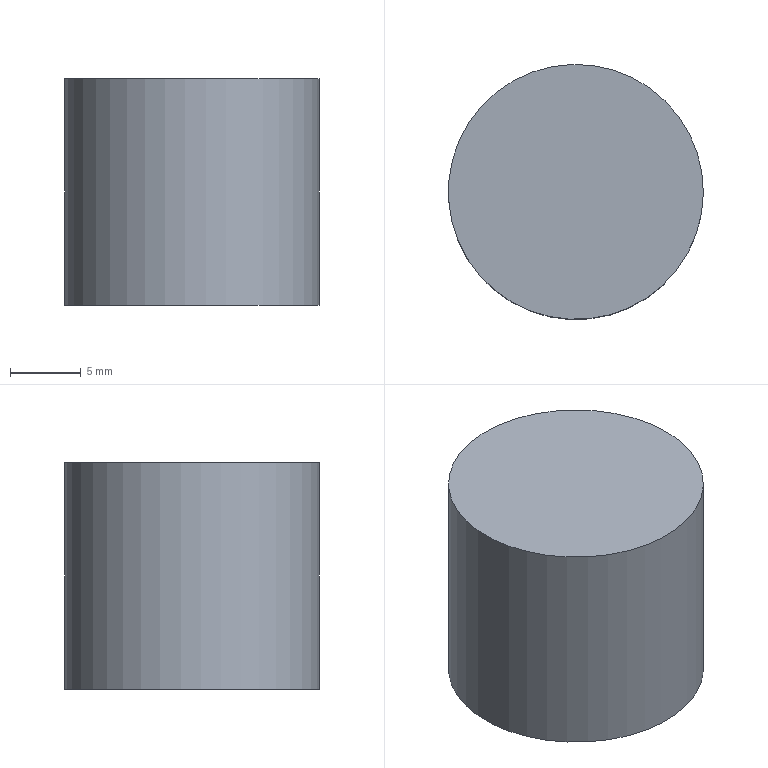Component | NX | PLUG | 1 solid | 3 faces | box 18 x 18 x 16 mm | volume 4072 mm3 | plane 2 | cylinder 1 | commonest cylinder face diameters 18 x1
STEP:
#1=CARTESIAN_POINT('',(0.,0.,0.));
#2=DIRECTION('',(0.,0.,1.));
#3=DIRECTION('',(1.,0.,0.));
#4=AXIS2_PLACEMENT_3D('',#1,#2,#3);
#5=CARTESIAN_POINT('',(72.936,-120.097,-169.615));
#6=VERTEX_POINT('',#5);
#7=CARTESIAN_POINT('',(81.249,-116.649,-169.615));
#8=DIRECTION('',(0.,0.,1.));
#9=DIRECTION('',(-0.9237,-0.383,0.));
#10=AXIS2_PLACEMENT_3D('',#7,#8,#9);
#11=CIRCLE('',#10,9.);
#12=CARTESIAN_POINT('',(81.249,-116.649,-169.615));
#13=DIRECTION('',(0.,0.,-1.));
#14=DIRECTION('',(-0.9237,-0.383,0.));
#15=AXIS2_PLACEMENT_3D('',#12,#13,#14);
#16=PLANE('',#15);
#17=CARTESIAN_POINT('',(9.,0.));
#18=CARTESIAN_POINT('',(9.,-15.588));
#19=CARTESIAN_POINT('',(-4.5,-7.794));
#20=CARTESIAN_POINT('',(-18.,-0.));
#21=CARTESIAN_POINT('',(-4.5,7.794));
#22=CARTESIAN_POINT('',(9.,15.588));
#23=CARTESIAN_POINT('',(9.,0.));
#24=(BOUNDED_CURVE()B_SPLINE_CURVE(2,(#17,#18,#19,#20,#21,#22,#23),.UNSPECIFIED.,.T.,.F.)B_SPLINE_CURVE_WITH_KNOTS((1,2,2,2,2,1),(-2.094,0.,2.094,4.189,6.283,8.378),.UNSPECIFIED.)CURVE()GEOMETRIC_REPRESENTATION_ITEM()RATIONAL_B_SPLINE_CURVE((1.,0.5,1.,0.5,1.,0.5,1.))REPRESENTATION_ITEM(''));
#25=(GEOMETRIC_REPRESENTATION_CONTEXT(2)PARAMETRIC_REPRESENTATION_CONTEXT()REPRESENTATION_CONTEXT('',''));
#26=DEFINITIONAL_REPRESENTATION('',(#24),#25);
#27=PCURVE('',#16,#26);
#28=CARTESIAN_POINT('',(81.249,-116.649,-153.615));
#29=DIRECTION('',(0.,0.,-1.));
#30=DIRECTION('',(-0.9237,-0.383,0.));
#31=AXIS2_PLACEMENT_3D('',#28,#29,#30);
#32=CYLINDRICAL_SURFACE('',#31,9.);
#33=CARTESIAN_POINT('',(6.283,16.));
#34=DIRECTION('',(-1.,0.));
#35=VECTOR('',#34,1.);
#36=LINE('',#33,#35);
#37=(GEOMETRIC_REPRESENTATION_CONTEXT(2)PARAMETRIC_REPRESENTATION_CONTEXT()REPRESENTATION_CONTEXT('',''));
#38=DEFINITIONAL_REPRESENTATION('',(#36),#37);
#39=PCURVE('',#32,#38);
#40=SURFACE_CURVE('',#11,(#27,#39),.PCURVE_S1.);
#41=EDGE_CURVE('',#6,#6,#40,.T.);
#42=ORIENTED_EDGE('',*,*,#41,.F.);
#43=EDGE_LOOP('',(#42));
#44=FACE_BOUND('',#43,.T.);
#45=ADVANCED_FACE('',(#44),#16,.T.);
#46=CARTESIAN_POINT('',(72.936,-120.097,-153.615));
#47=VERTEX_POINT('',#46);
#48=CARTESIAN_POINT('',(81.249,-116.649,-153.615));
#49=DIRECTION('',(0.,0.,-1.));
#50=DIRECTION('',(-0.9237,-0.383,0.));
#51=AXIS2_PLACEMENT_3D('',#48,#49,#50);
#52=CIRCLE('',#51,9.);
#53=CARTESIAN_POINT('',(81.249,-116.649,-153.615));
#54=DIRECTION('',(0.,0.,1.));
#55=DIRECTION('',(0.9237,0.383,0.));
#56=AXIS2_PLACEMENT_3D('',#53,#54,#55);
#57=PLANE('',#56);
#58=CARTESIAN_POINT('',(-9.,0.));
#59=CARTESIAN_POINT('',(-9.,15.588));
#60=CARTESIAN_POINT('',(4.5,7.794));
#61=CARTESIAN_POINT('',(18.,0.));
#62=CARTESIAN_POINT('',(4.5,-7.794));
#63=CARTESIAN_POINT('',(-9.,-15.588));
#64=CARTESIAN_POINT('',(-9.,0.));
#65=(BOUNDED_CURVE()B_SPLINE_CURVE(2,(#58,#59,#60,#61,#62,#63,#64),.UNSPECIFIED.,.T.,.F.)B_SPLINE_CURVE_WITH_KNOTS((1,2,2,2,2,1),(-2.094,0.,2.094,4.189,6.283,8.378),.UNSPECIFIED.)CURVE()GEOMETRIC_REPRESENTATION_ITEM()RATIONAL_B_SPLINE_CURVE((1.,0.5,1.,0.5,1.,0.5,1.))REPRESENTATION_ITEM(''));
#66=(GEOMETRIC_REPRESENTATION_CONTEXT(2)PARAMETRIC_REPRESENTATION_CONTEXT()REPRESENTATION_CONTEXT('',''));
#67=DEFINITIONAL_REPRESENTATION('',(#65),#66);
#68=PCURVE('',#57,#67);
#69=CARTESIAN_POINT('',(0.,0.));
#70=DIRECTION('',(1.,0.));
#71=VECTOR('',#70,1.);
#72=LINE('',#69,#71);
#73=(GEOMETRIC_REPRESENTATION_CONTEXT(2)PARAMETRIC_REPRESENTATION_CONTEXT()REPRESENTATION_CONTEXT('',''));
#74=DEFINITIONAL_REPRESENTATION('',(#72),#73);
#75=PCURVE('',#32,#74);
#76=SURFACE_CURVE('',#52,(#68,#75),.PCURVE_S1.);
#77=EDGE_CURVE('',#47,#47,#76,.T.);
#78=ORIENTED_EDGE('',*,*,#77,.F.);
#79=EDGE_LOOP('',(#78));
#80=FACE_BOUND('',#79,.T.);
#81=ADVANCED_FACE('',(#80),#57,.T.);
#82=ORIENTED_EDGE('',*,*,#41,.T.);
#83=CARTESIAN_POINT('',(72.936,-120.097,-153.615));
#84=CARTESIAN_POINT('',(72.936,-120.097,-169.615));
#85=B_SPLINE_CURVE_WITH_KNOTS('',1,(#83,#84),.UNSPECIFIED.,.F.,.F.,(2,2),(0.,16.),.PIECEWISE_BEZIER_KNOTS.);
#86=CARTESIAN_POINT('',(0.,0.));
#87=DIRECTION('',(0.,1.));
#88=VECTOR('',#87,1.);
#89=LINE('',#86,#88);
#90=(GEOMETRIC_REPRESENTATION_CONTEXT(2)PARAMETRIC_REPRESENTATION_CONTEXT()REPRESENTATION_CONTEXT('',''));
#91=DEFINITIONAL_REPRESENTATION('',(#89),#90);
#92=PCURVE('',#32,#91);
#93=CARTESIAN_POINT('',(6.283,0.));
#94=DIRECTION('',(0.,1.));
#95=VECTOR('',#94,1.);
#96=LINE('',#93,#95);
#97=(GEOMETRIC_REPRESENTATION_CONTEXT(2)PARAMETRIC_REPRESENTATION_CONTEXT()REPRESENTATION_CONTEXT('',''));
#98=DEFINITIONAL_REPRESENTATION('',(#96),#97);
#99=PCURVE('',#32,#98);
#100=SEAM_CURVE('',#85,(#92,#99),.PCURVE_S1.);
#101=EDGE_CURVE('',#47,#6,#100,.T.);
#102=ORIENTED_EDGE('',*,*,#101,.F.);
#103=ORIENTED_EDGE('',*,*,#77,.T.);
#104=ORIENTED_EDGE('',*,*,#101,.T.);
#105=EDGE_LOOP('',(#82,#102,#103,#104));
#106=FACE_BOUND('',#105,.T.);
#107=ADVANCED_FACE('',(#106),#32,.T.);
#108=CLOSED_SHELL('',(#45,#81,#107));
#109=MANIFOLD_SOLID_BREP('',#108);
#110=(LENGTH_UNIT()NAMED_UNIT(*)SI_UNIT(.MILLI.,.METRE.));
#111=UNCERTAINTY_MEASURE_WITH_UNIT(LENGTH_MEASURE(0.00001),#110,'','');
#112=(NAMED_UNIT(*)PLANE_ANGLE_UNIT()SI_UNIT($,.RADIAN.));
#113=(NAMED_UNIT(*)SI_UNIT($,.STERADIAN.)SOLID_ANGLE_UNIT());
#114=(GEOMETRIC_REPRESENTATION_CONTEXT(3)GLOBAL_UNCERTAINTY_ASSIGNED_CONTEXT((#111))GLOBAL_UNIT_ASSIGNED_CONTEXT((#110,#112,#113))REPRESENTATION_CONTEXT('',''));
#115=ADVANCED_BREP_SHAPE_REPRESENTATION('',(#4,#109),#114);